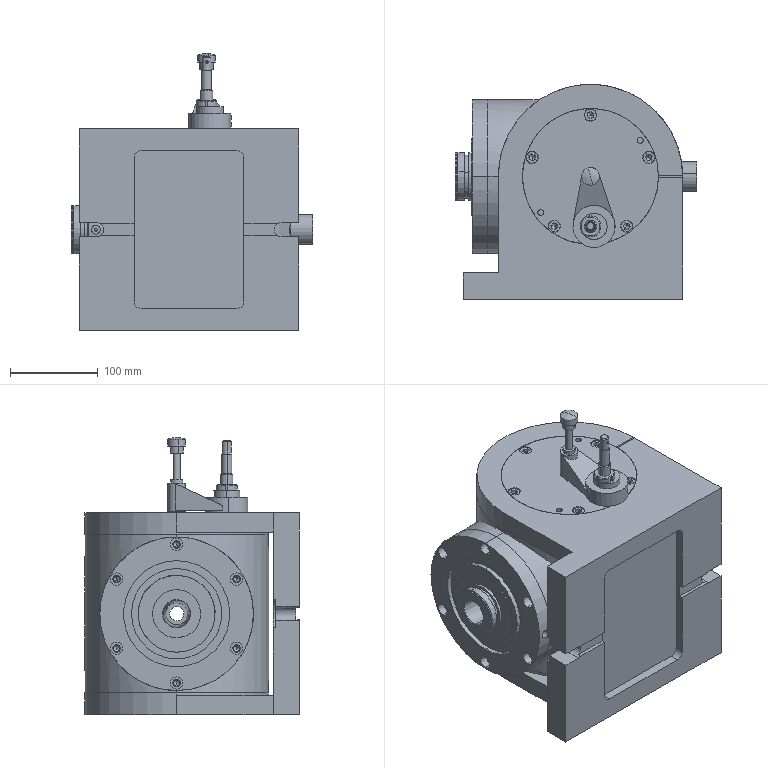Assembly | SolidWorks | mm | 42 component files | 42 solids | 5216 faces | box 275 x 245 x 316 mm | volume 7786043 mm3 | cylinder 1911 | plane 1680 | spline 1262 | cone 213 | torus 148 | sphere 2 | commonest cylinder face diameters 120 x604 115.5 x472 124.5 x122 96 x120 8 x68 14 x46 10 x40 8.5 x36
Bill of materials:
10HexSocketScrewM8X25 | 4 |  | Headed cylindrical fastener-like part: short cylindrical head with a hexagonal socket recess and a long plain cylindrical shank with a chamfered tip.
11Base | 1 |  | C-shaped split-clamp bracket: two parallel plates, each with a large circular bore and a thin radial split, joined by a rectangular back wall with a foot flange at the base.
12Turbine | 1 |  | Long slender stepped shaft with several diameter steps, a small cross hole near the narrow end, a band of closely spaced circumferential/helical grooves in the middle, and a larger collar and flange at the base.
13EccentricSleeve | 1 |  | Stepped hollow cylindrical sleeve: a smaller-diameter tube on top of a larger-diameter body, with a through bore and a rounded-end side cutout on the larger section.
14FrontFlange | 1 |  | Thick circular disc/plate with a ring of through holes near the rim, a small central hole or spot, and one large off-center hole with an edge chamfer or counterbore.
15Lever | 1 |  | Lever/crank arm: a large ring hub with a big bore connected by a tapered web to a smaller boss with a small bore; the boss sits at a different height from the hub.
16RoundNutM14X1.5 | 1 |  | Thick annular ring with four equally spaced rectangular slots in the outer edge and chamfers on both outer edges.
17Handle | 1 |  | Knob or cap-like part: a cylindrical head with a slightly domed top on a smaller cylindrical stem that has a transverse hole.
18Pin | 1 |  | Cylindrical pin with an integral collar near one end, a small cross hole near the other end, and chamfered ends.
19LockNut | 1 |  | Thin flat ring/washer with four small rectangular notches on the outer edge at 90-degree spacing.
1Turbine | 1 |  | Flanged cylindrical bushing with a through bore, a relief neck under the flange, a knurled/serrated band, and a short pilot step at the end.
20Gear | 2 |  | Ring with two thin rims of fine external teeth on either face, separated by a smaller-diameter central band, with a large plain bore.
21Spacer | 1 |  | Narrow plain annular ring with rectangular cross-section and one small radial hole through the wall.
22Bushing | 1 |  | Thin-walled cylindrical sleeve or tube, longer axially than its diameter, with a single small radial hole in the wall.
23RingGear | 1 |  | Ring with a smooth cylindrical outside surface and a full circle of many small straight teeth around the inner bore; looks like an internal gear or internally splined ring.
24Gasket | 1 |  | Thin flat washer-like ring with a raised annular step around the bore on one face and chamfered or angled outer edges.
25SealRing | 1 |  | Very thin plain flat ring (shim- or gasket-like annulus) with a narrow radial width.
26TaperSleeve | 1 |  | Flanged annular cover or housing plate: a wide flat flange with six evenly spaced axial through holes, two stepped concentric bosses on one face, a large central bore with an axial slot in it, and a small hole in the outer rim.
27Spindle | 1 |  | Stepped, turned shaft with a tapered (conical) section near the large end, several cylindrical steps that get smaller toward the other end, an elongated keyway slot on one step, small grooves near the large end, and a central bore at the small end.
28ParallelKey8X32 | 1 |  | Solid elongated bar with a stadium-shaped (rounded-end) outline and slightly rounded edges; shaped like a round-ended parallel key.
2InsulatingRing | 2 |  | Flat ring with a one-step profile (thinner outer flange and a thicker inner portion on one face) and a small tab or notch at the bore.
3CopperRing | 1 |  | Plain cylindrical ring or sleeve with a rectangular cross-section, moderate axial width and a thin wall, with no visible extra features.
4RoundNutM52X1.5 | 1 |  | Thick annular ring with chamfered outer edges and four evenly spaced rectangular slots cut into the outer edge, giving a slotted round-nut-like shape.
5ThrustWasher | 1 |  | Plain flat annular ring or thick washer with a rectangular cross-section and a relatively wide radial wall.
6Bushing | 1 |  | Flanged cylindrical sleeve: a thin circular flange with four through-holes, joined to a coaxial cylindrical hub with a large central through-bore and one small radial hole in the hub wall.
7 | 1 |  | Cylindrical housing body with a partial cylindrical boss crossing it on one side. Its top face has an irregular cavity with several bores and small holes. One side face has a flat-bottomed spot face with a central bore and four holes around it, and there are smaller notches and cutouts on the outer wall.
8RearFlange | 1 |  | Short disc or ring-shaped plate with a shallow pocket on one face. The pocket wall has a scalloped, irregular contour. There is one larger through-hole off the centre and seven smaller holes near the outer edge.
9HexSocketScrewM8X35 | 10 |  | Headed cylindrical pin or screw-like shape: a short, larger-diameter cylindrical head with a long, smooth, coaxial cylindrical shank that has a chamfer at its free end.
Mates:
1. concentric | 11Base-1 face at (33.957, 1.776, 135) dir (0, 0, 1) r 77.5 | 7-1 face at (33.957, 1.776, 340) dir (0, 0, -1) r 105
2. coincident | 11Base-1 face at (33.957, 1.776, 340) dir (0, 0, -1) | 7-1 face at (33.957, 1.776, 340) dir (0, 0, 1)
3. concentric | 7-1 face at (138.958, 1.776, 250) dir (-1, 0, 0) r 87.5 | 26TaperSleeve-1 face at (-65.043, 1.776, 250) dir (1, 0, 0) r 87.5
4. concentric | 7-1 face at (-83.043, 70.192, 210.5) dir (-1, 0, 0) r 3.4 | 26TaperSleeve-1 face at (-92.043, 70.192, 210.5) dir (-1, 0, 0) r 7
5. concentric | 25SealRing-1 face at (-63.543, 1.776, 250) dir (-1, 0, 0) r 36 | 24Gasket-1 face at (-61.043, 1.776, 250) dir (1, 0, 0) r 36
6. coincident | 25SealRing-1 face at (-63.543, 1.776, 250) dir (1, 0, 0) | 24Gasket-1 face at (-63.543, 45.776, 250) dir (-1, 0, 0)
7. concentric | 27Spindle-1 face at (-13.043, 1.776, 250) dir (-1, 0, 0) r 32.5 | 25SealRing-1 face at (-63.543, 1.776, 250) dir (-1, 0, 0) r 36
8. coincident | 27Spindle-1 face at (-65.043, 1.776, 250) dir (1, 0, 0) | 25SealRing-1 face at (-65.043, 1.776, 250) dir (-1, 0, 0)
9. concentric | 27Spindle-1 face at (-13.043, 1.776, 250) dir (-1, 0, 0) r 32.5 | 22Bushing-1 face at (-10.043, 1.776, 250) dir (-1, 0, 0) r 37.5
10. coincident | 27Spindle-1 face at (-60.043, 1.776, 250) dir (1, 0, 0) | 22Bushing-1 face at (-60.043, 1.776, 250) dir (-1, 0, 0)
11. concentric | 22Bushing-1 face at (-10.043, 1.776, 250) dir (-1, 0, 0) r 37.5 | 20Gear-1 face at (-55.043, 1.776, 250) dir (1, 0, 0) r 45
12. coincident | 22Bushing-1 edge at (-60.043, 1.776, 250) dir (1, 0, 0) r 37.5 | 20Gear-1 face at (-60.043, 1.776, 250) dir (-1, 0, 0)
13. concentric | 22Bushing-1 face at (-10.043, 1.776, 250) dir (-1, 0, 0) r 37.5 | 21Spacer-1 face at (-30.043, 1.776, 250) dir (-1, 0, 0) r 45
14. coincident | 20Gear-1 face at (-40.043, 1.776, 250) dir (1, 0, 0) | 21Spacer-1 face at (-40.043, 1.776, 250) dir (-1, 0, 0)
15. concentric | 22Bushing-1 face at (-10.043, 1.776, 250) dir (-1, 0, 0) r 37.5 | 20Gear-2 face at (-25.043, 1.776, 250) dir (1, 0, 0) r 45
16. coincident | 21Spacer-1 face at (-30.043, 1.776, 250) dir (1, 0, 0) | 20Gear-2 face at (-30.043, 1.776, 250) dir (-1, 0, 0)
17. concentric | 27Spindle-1 face at (72.957, 1.776, 250) dir (-1, 0, 0) r 27.5 | 23RingGear-1 face at (-10.043, 1.776, 250) dir (-1, 0, 0) r 72.5
18. concentric | 27Spindle-1 face at (72.957, 1.776, 250) dir (-1, 0, 0) r 27.5 | 19LockNut-1 face at (-4.043, 1.776, 250) dir (1, 0, 0) r 32
19. coincident | 22Bushing-1 face at (-10.043, 1.776, 250) dir (1, 0, 0) | 19LockNut-1 face at (-10.043, 1.776, 250) dir (-1, 0, 0)
20. concentric | 27Spindle-1 face at (72.957, 1.776, 250) dir (-1, 0, 0) r 27.5 | 1Turbine-1 face at (-3.043, 1.776, 250) dir (1, 0, 0) r 27.5
21. coincident | 27Spindle-1 face at (10.957, -21.064, 250.765) dir (0, 0.2079, 0.9781) | 28ParallelKey8X32-1 face at (10.957, -21.064, 250.765) dir (0, -0.2079, -0.9781)
22. concentric | 27Spindle-1 face at (34.957, -20.232, 254.678) dir (0, -0.9781, 0.2079) r 4 | 28ParallelKey8X32-1 face at (34.957, -20.232, 254.678) dir (0, -0.9781, 0.2079) r 4
23. coincident | 27Spindle-1 face at (10.957, -20.232, 254.678) dir (0, -0.9781, 0.2079) | 28ParallelKey8X32-1 face at (10.957, -20.232, 254.678) dir (0, 0.9781, -0.2079)
24. parallel | 1Turbine-1 face at (-3.043, -27.666, 256.258) dir (0, 0.9781, -0.2079) | 28ParallelKey8X32-1 face at (10.957, -26.59, 256.029) dir (0, -0.9781, 0.2079)
25. coincident | 27Spindle-1 face at (-3.043, 1.776, 250) dir (1, 0, 0) | 1Turbine-1 face at (-3.043, 1.776, 250) dir (-1, 0, 0)
26. concentric | 27Spindle-1 face at (154.957, 1.776, 250) dir (-1, 0, 0) r 17 | 2InsulatingRing-1 face at (18.957, 1.776, 250) dir (1, 0, 0) r 27.5
27. concentric | 27Spindle-1 face at (154.957, 1.776, 250) dir (-1, 0, 0) r 17 | 3CopperRing-1 face at (48.957, 1.776, 250) dir (1, 0, 0) r 34
28. concentric | 27Spindle-1 face at (154.957, 1.776, 250) dir (-1, 0, 0) r 17 | 2InsulatingRing-2 face at (100.957, 1.776, 250) dir (-1, 0, 0) r 27.5
29. coincident | 2InsulatingRing-1 face at (48.957, 1.776, 250) dir (1, 0, 0) | 3CopperRing-1 face at (48.957, 1.776, 250) dir (-1, 0, 0)
30. coincident | 3CopperRing-1 face at (70.957, 1.776, 250) dir (1, 0, 0) | 2InsulatingRing-2 face at (70.957, 1.776, 250) dir (-1, 0, 0)
31. coincident | 1Turbine-1 face at (46.957, 1.776, 250) dir (1, 0, 0) | 2InsulatingRing-1 face at (46.957, 1.776, 250) dir (-1, 0, 0)
32. concentric | 3CopperRing-1 face at (48.957, 1.776, 250) dir (1, 0, 0) r 40 | 4RoundNutM52X1.5-1 face at (72.957, 1.776, 250) dir (-1, 0, 0) r 26
33. coincident | 2InsulatingRing-2 face at (72.957, 1.776, 250) dir (1, 0, 0) | 4RoundNutM52X1.5-1 face at (72.957, 1.776, 250) dir (-1, 0, 0)
34. concentric | 27Spindle-1 face at (154.957, 1.776, 250) dir (-1, 0, 0) r 17 | 5ThrustWasher-1 face at (95.957, 1.776, 250) dir (-1, 0, 0) r 30
35. coincident | 4RoundNutM52X1.5-1 face at (87.957, 1.776, 250) dir (1, 0, 0) | 5ThrustWasher-1 face at (87.957, 1.776, 250) dir (-1, 0, 0)
36. concentric | 27Spindle-1 face at (154.957, 1.776, 250) dir (-1, 0, 0) r 17 | 6Bushing-1 face at (80.387, 1.776, 250) dir (-1, 0, 0) r 21
37. coincident | 5ThrustWasher-1 face at (95.957, 1.776, 250) dir (1, 0, 0) | 6Bushing-1 face at (95.957, 1.776, 292.5) dir (-1, 0, 0)
38. concentric | 26TaperSleeve-1 face at (-65.043, 1.776, 250) dir (1, 0, 0) r 87.5 | 27Spindle-1 face at (-102.043, 1.776, 250) dir (1, 0, 0) r 174.533
39. coincident | 7-1 face at (-83.043, 1.776, 250) dir (-1, 0, 0) | 26TaperSleeve-1 face at (-83.043, 89.276, 250) dir (1, 0, 0)
40. parallel | 11Base-1 face at (13.957, -108.224, 250) dir (0, 1, 0) | 7-1 face at (33.957, 73.776, 325) dir (0, 1, 0)
41. coincident | 26TaperSleeve-1 face at (-65.043, 51.776, 250) dir (1, 0, 0) | 24Gasket-1 face at (-65.043, 54.276, 250) dir (-1, 0, 0)
42. coincident | 20Gear-1 face at (-60.043, 1.776, 250) dir (-1, 0, 0) | 23RingGear-1 face at (-60.043, 1.776, 250) dir (-1, 0, 0)
43. concentric | 7-1 face at (33.957, 71.776, 170) dir (0, 0, -1) r 4 | 9HexSocketScrewM8X35-1 face at (33.957, 71.776, 179) dir (0, 0, -1) r 4
44. concentric | 7-1 face at (100.531, 23.407, 330) dir (0, 0, 1) r 4 | 9HexSocketScrewM8X35-6 face at (100.531, 23.407, 321) dir (0, 0, 1) r 4
45. concentric | 11Base-1 face at (33.957, 1.776, 135) dir (0, 0, 1) r 77.5 | 8RearFlange-1 face at (33.957, 1.776, 170) dir (0, 0, -1) r 77.5
46. concentric | 7-1 face at (6.957, 1.776, 155) dir (0, 0, 1) r 15 | 8RearFlange-1 face at (6.957, 1.776, 135) dir (0, 0, 1) r 15
47. coincident | 9HexSocketScrewM8X35-1 face at (33.957, 71.776, 144) dir (0, 0, 1) | 8RearFlange-1 face at (33.957, 71.776, 144) dir (0, 0, -1)
48. coincident | 7-1 face at (33.957, 1.776, 170) dir (0, 0, -1) | 8RearFlange-1 face at (33.957, 1.776, 170) dir (0, 0, 1)
49. concentric | 12Turbine-1 face at (33.957, -55.224, 386) dir (0, 0, -1) r 7.5 | 13EccentricSleeve-1 face at (33.957, -55.224, 290) dir (0, 0, -1) r 13.75
50. coincident | 12Turbine-1 face at (33.957, -55.224, 190) dir (0, 0, 1) | 13EccentricSleeve-1 face at (37.957, -55.224, 190) dir (0, 0, -1)
51. concentric | 7-1 face at (37.957, -55.224, 340) dir (0, 0, -1) r 20 | 13EccentricSleeve-1 face at (37.957, -55.224, 330) dir (0, 0, -1) r 20
52. concentric | 11Base-1 face at (33.957, 1.776, 135) dir (0, 0, 1) r 77.5 | 14FrontFlange-1 face at (33.957, 1.776, 330) dir (0, 0, 1) r 77.5
53. concentric | 13EccentricSleeve-1 face at (37.957, -55.224, 390) dir (0, 0, -1) r 15 | 14FrontFlange-1 face at (37.957, -55.224, 365) dir (0, 0, -1) r 15
54. coincident | 9HexSocketScrewM8X35-7 face at (33.957, 71.776, 356) dir (0, 0, -1) | 14FrontFlange-1 face at (33.957, 71.776, 356) dir (0, 0, 1)
55. coincident | 11Base-1 face at (-111.043, -108.224, 365) dir (0, 0, 1) | 14FrontFlange-1 face at (33.957, 1.776, 365) dir (0, 0, 1)
56. coincident | 14FrontFlange-1 face at (33.957, 1.776, 365) dir (0, 0, 1) | 15Lever-1 face at (37.957, -55.224, 365) dir (0, 0, -1)
57. concentric | 13EccentricSleeve-1 face at (37.957, -55.224, 390) dir (0, 0, -1) r 15 | 15Lever-1 face at (37.957, -55.224, 383) dir (0, 0, -1) r 24
58. concentric | 18Pin-1 face at (33.957, 1.776, 441) dir (0, 0, -1) r 4 | 17Handle-1 face at (33.957, 1.776, 433) dir (0, 0, -1) r 4
59. concentric | 18Pin-1 face at (32.89, 5.631, 437) dir (0.2668, -0.9637, 0) r 17.453 | 17Handle-1 face at (35.958, -5.452, 437) dir (-0.2668, 0.9637, 0) r 17.453
60. concentric | 15Lever-1 face at (33.957, 1.776, 365) dir (0, 0, 1) r 4.01 | 18Pin-1 face at (33.957, 1.776, 441) dir (0, 0, -1) r 4
61. coincident | 15Lever-1 face at (33.957, 1.776, 399) dir (0, 0, 1) | 18Pin-1 face at (33.957, 1.776, 399) dir (0, 0, -1)
62. concentric | 12Turbine-1 face at (33.957, -55.224, 410) dir (0, 0, -1) r 7 | 16RoundNutM14X1.5-1 face at (33.957, -55.224, 397) dir (0, 0, 1) r 7
63. coincident | 13EccentricSleeve-1 face at (37.957, -55.224, 390) dir (0, 0, 1) | 16RoundNutM14X1.5-1 face at (33.957, -55.224, 390) dir (0, 0, -1)
64. concentric | 7-1 face at (117.957, 26.525, 225.251) dir (1, 0, 0) r 7 | 10HexSocketScrewM8X25-1 face at (92.957, 26.525, 225.251) dir (1, 0, 0) r 4
65. coincident | 7-1 face at (117.957, 26.525, 225.251) dir (1, 0, 0) | 10HexSocketScrewM8X25-1 face at (117.957, 26.525, 225.251) dir (-1, 0, 0)
66. coincident | 13EccentricSleeve-1 face at (37.957, -55.224, 330) dir (0, 0, 1) | 14FrontFlange-1 face at (33.957, 1.776, 330) dir (0, 0, -1)
67. concentric | 14FrontFlange-1 face at (33.957, 1.776, 365) dir (0, 0, 1) r 4 | 18Pin-1 face at (33.957, 1.776, 441) dir (0, 0, -1) r 4
68. parallel | 7-1 face at (33.957, 73.776, 325) dir (0, 1, 0) | 13EccentricSleeve-1 plane at (37.957, -55.224, 190) dir (0, 1, 0)
69. gear | 1Turbine-1 sketch segment at (33.957, 1.776, 250) dir (1, 0, 0) r 45 | 12Turbine-1 sketch segment at (35.302, -67.148, 224.707) dir (0, 0, 1)